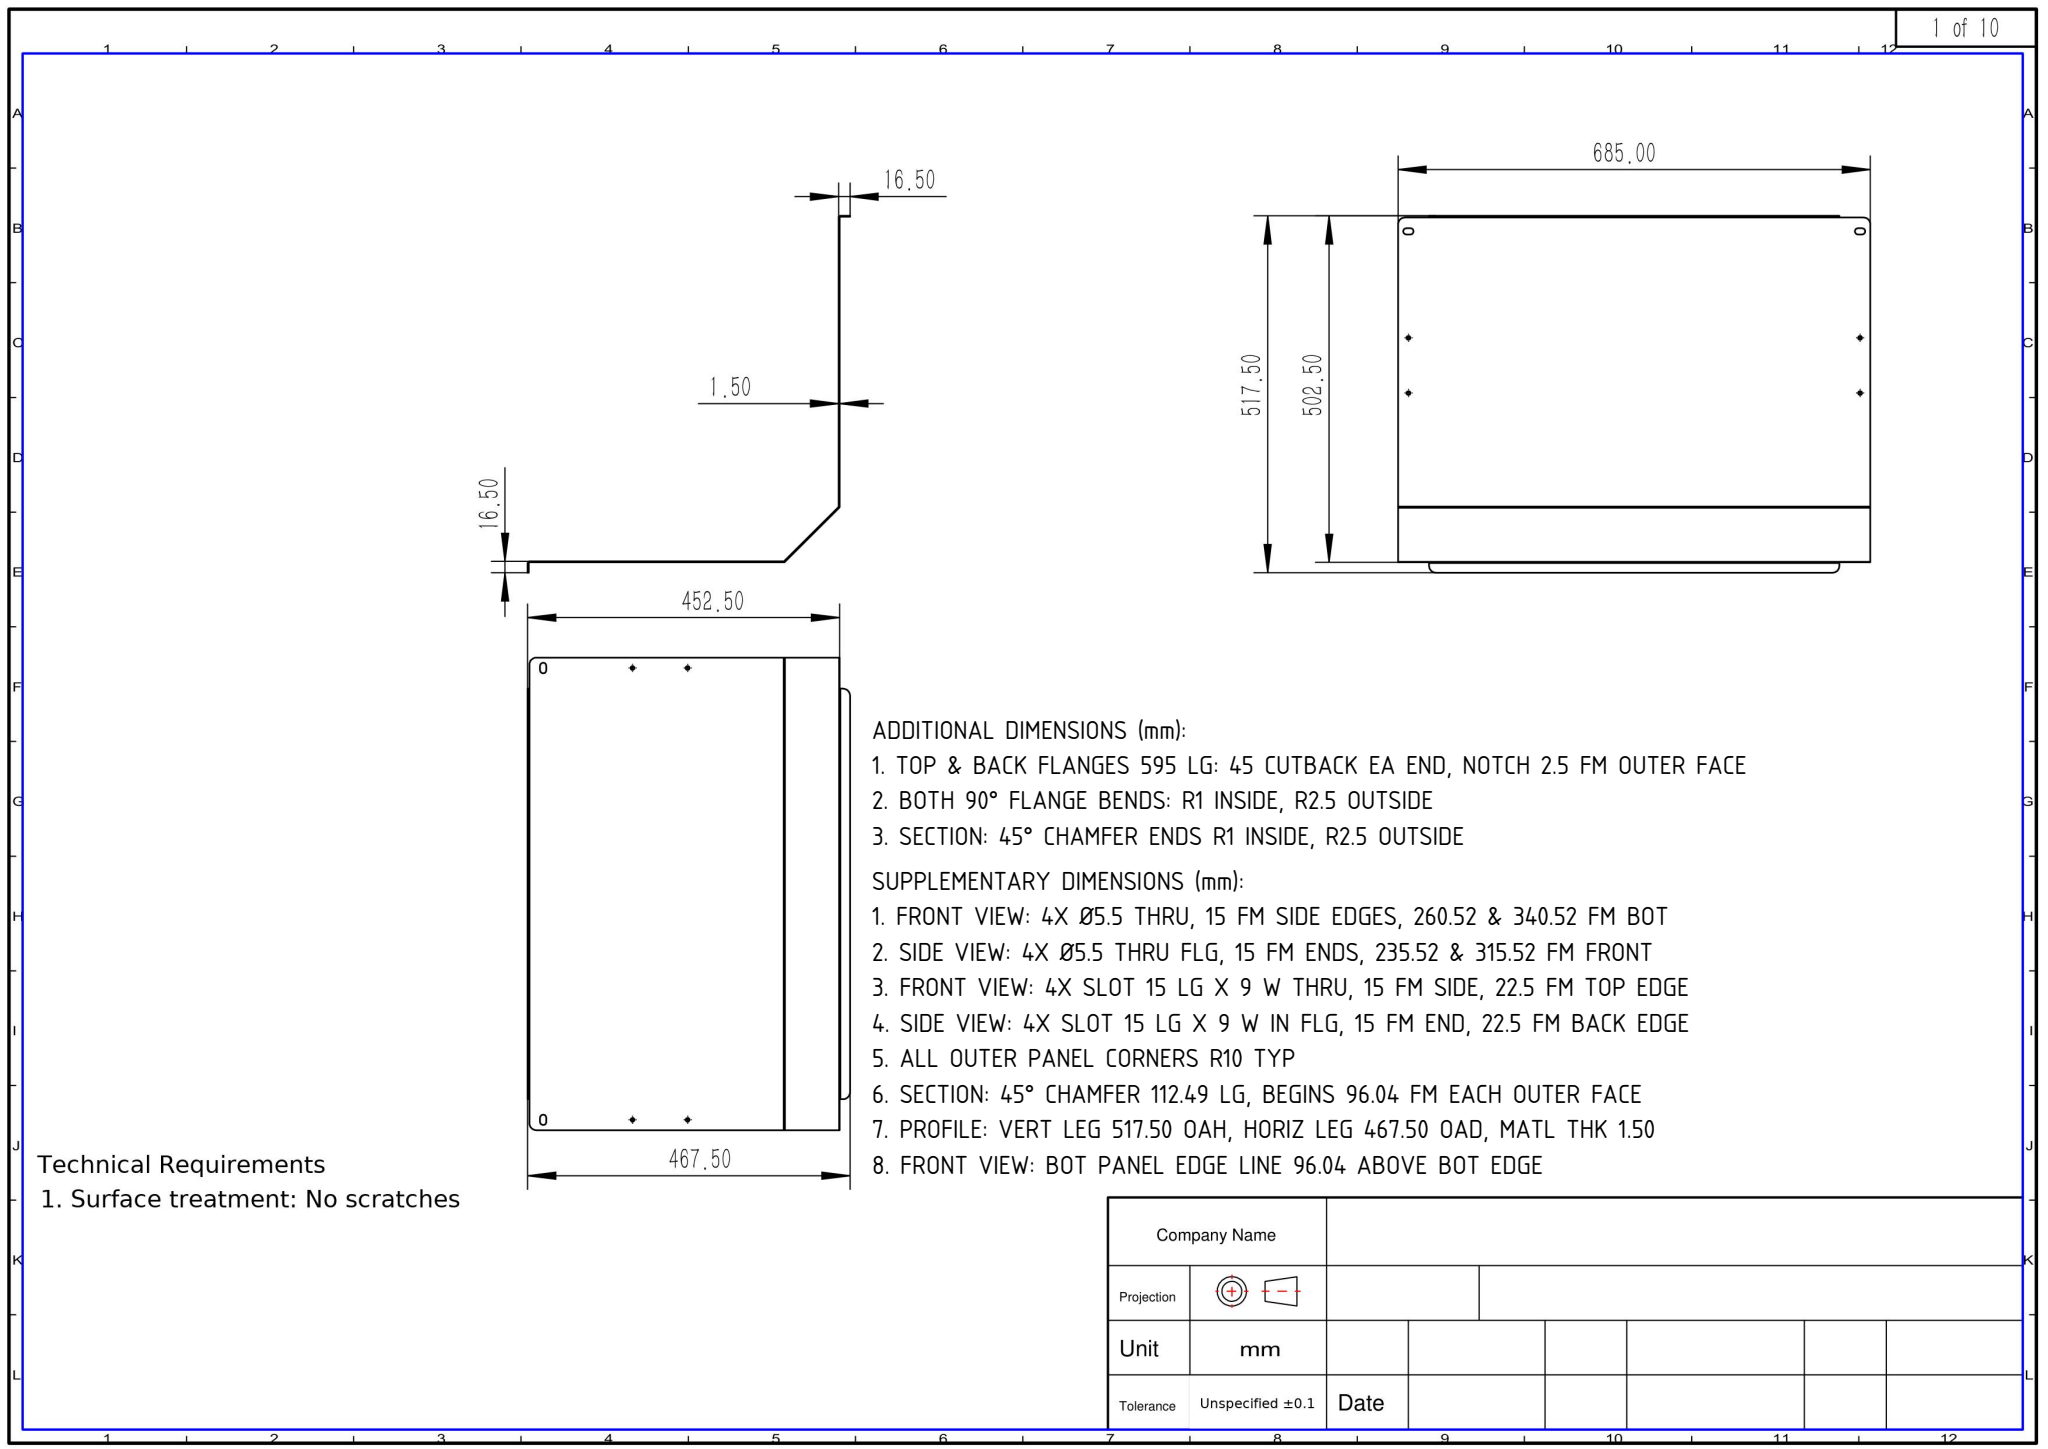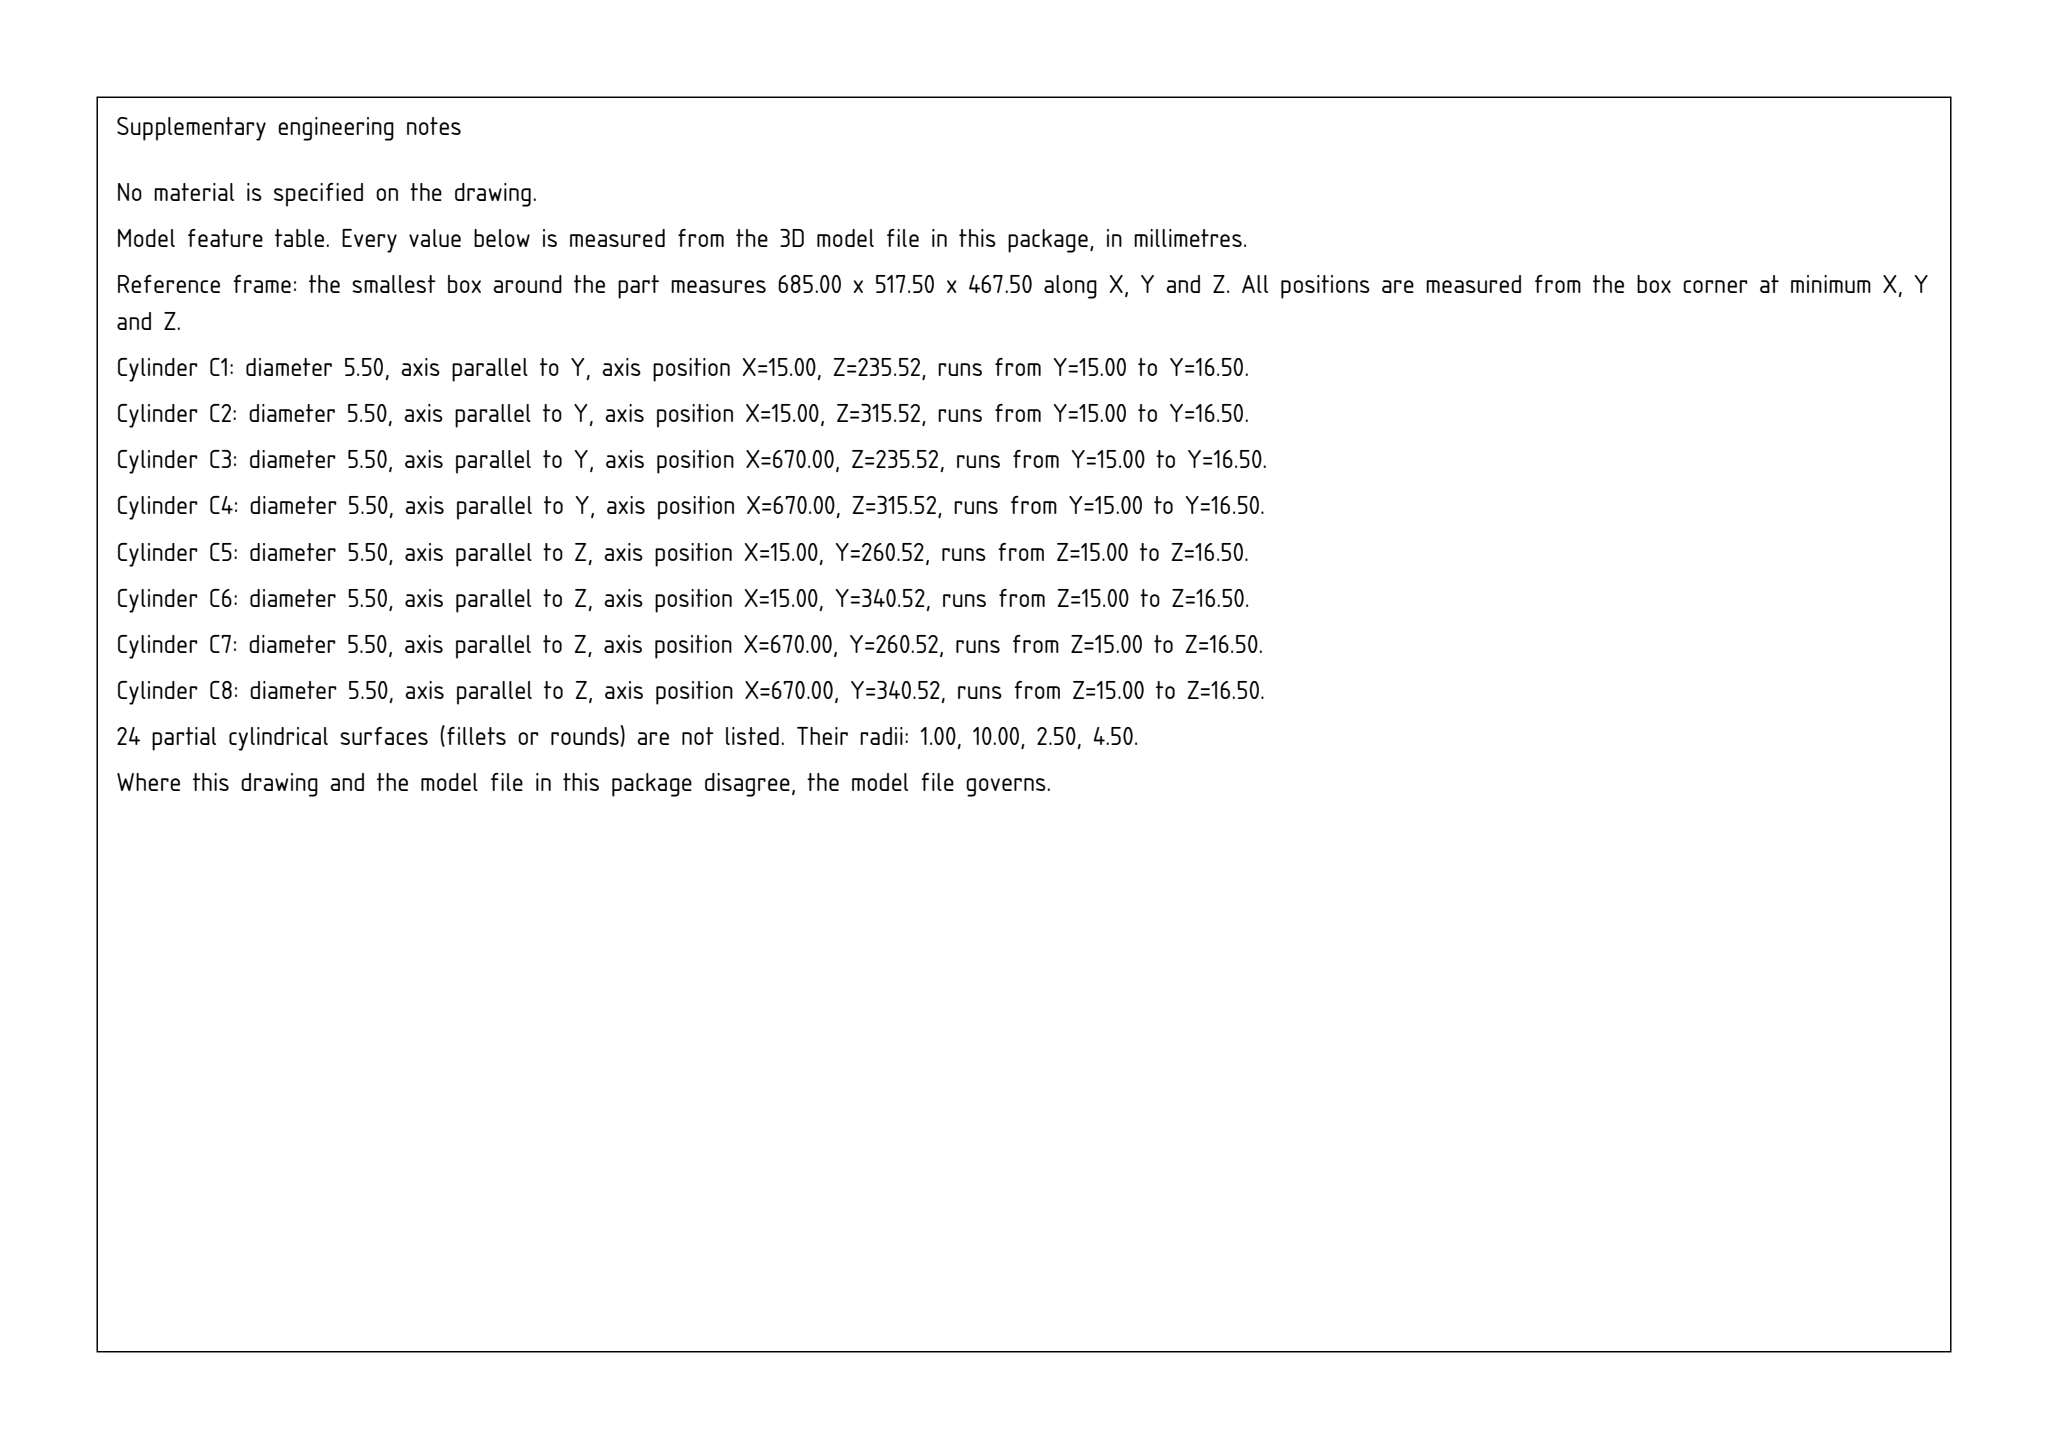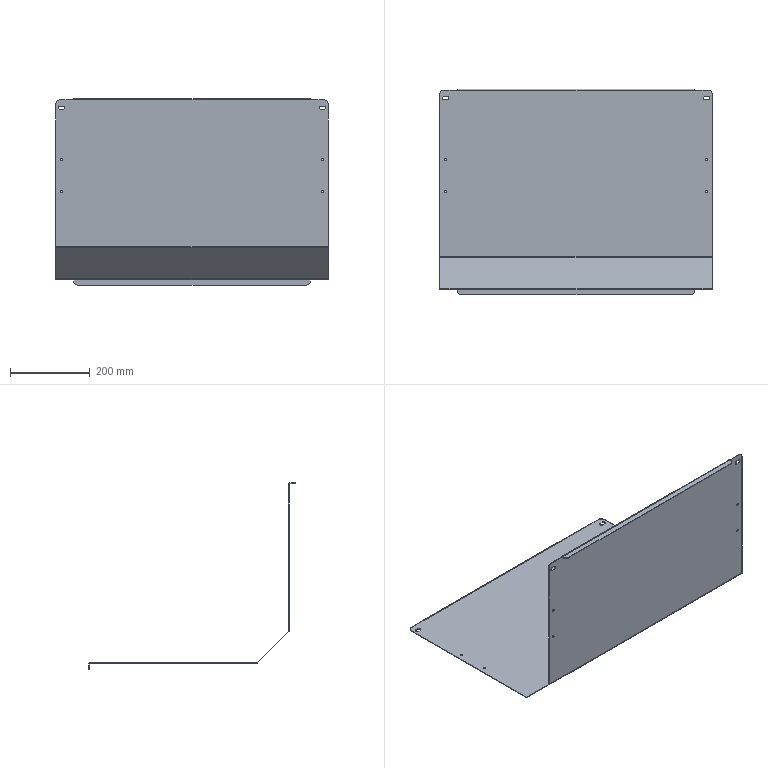Part | SolidWorks | mm | 1 solid | 84 faces | box 685 x 517.5 x 467.5 mm | volume 955190 mm3 | cylinder 42 | plane 42 | commonest cylinder face diameters 5.5 x16 9 x10 20 x8 2 x4 5 x4